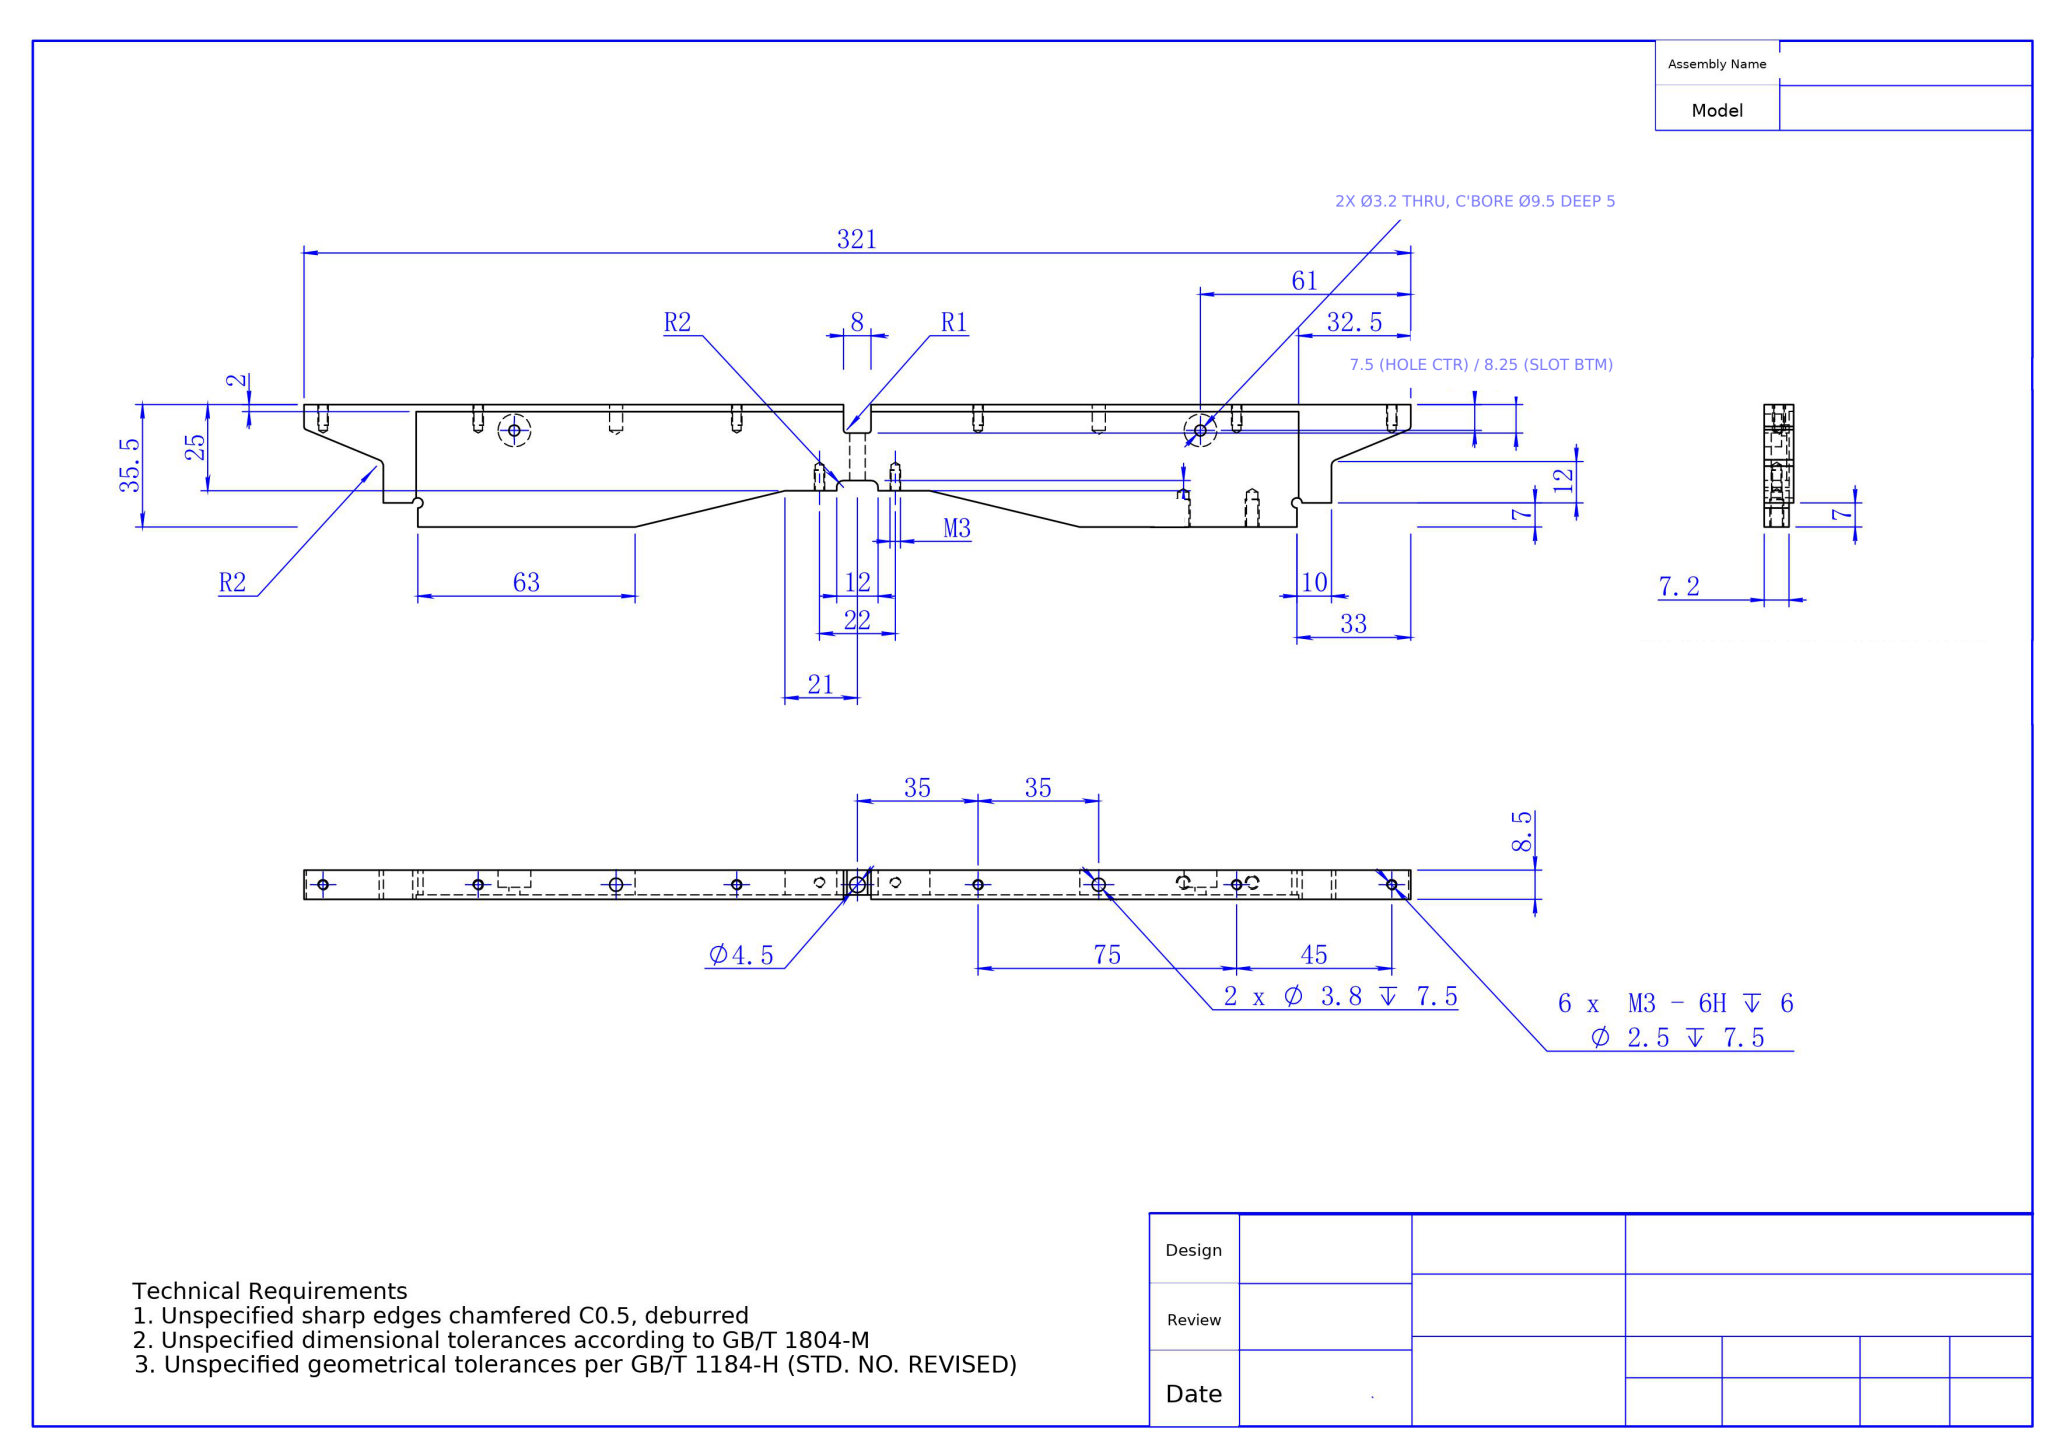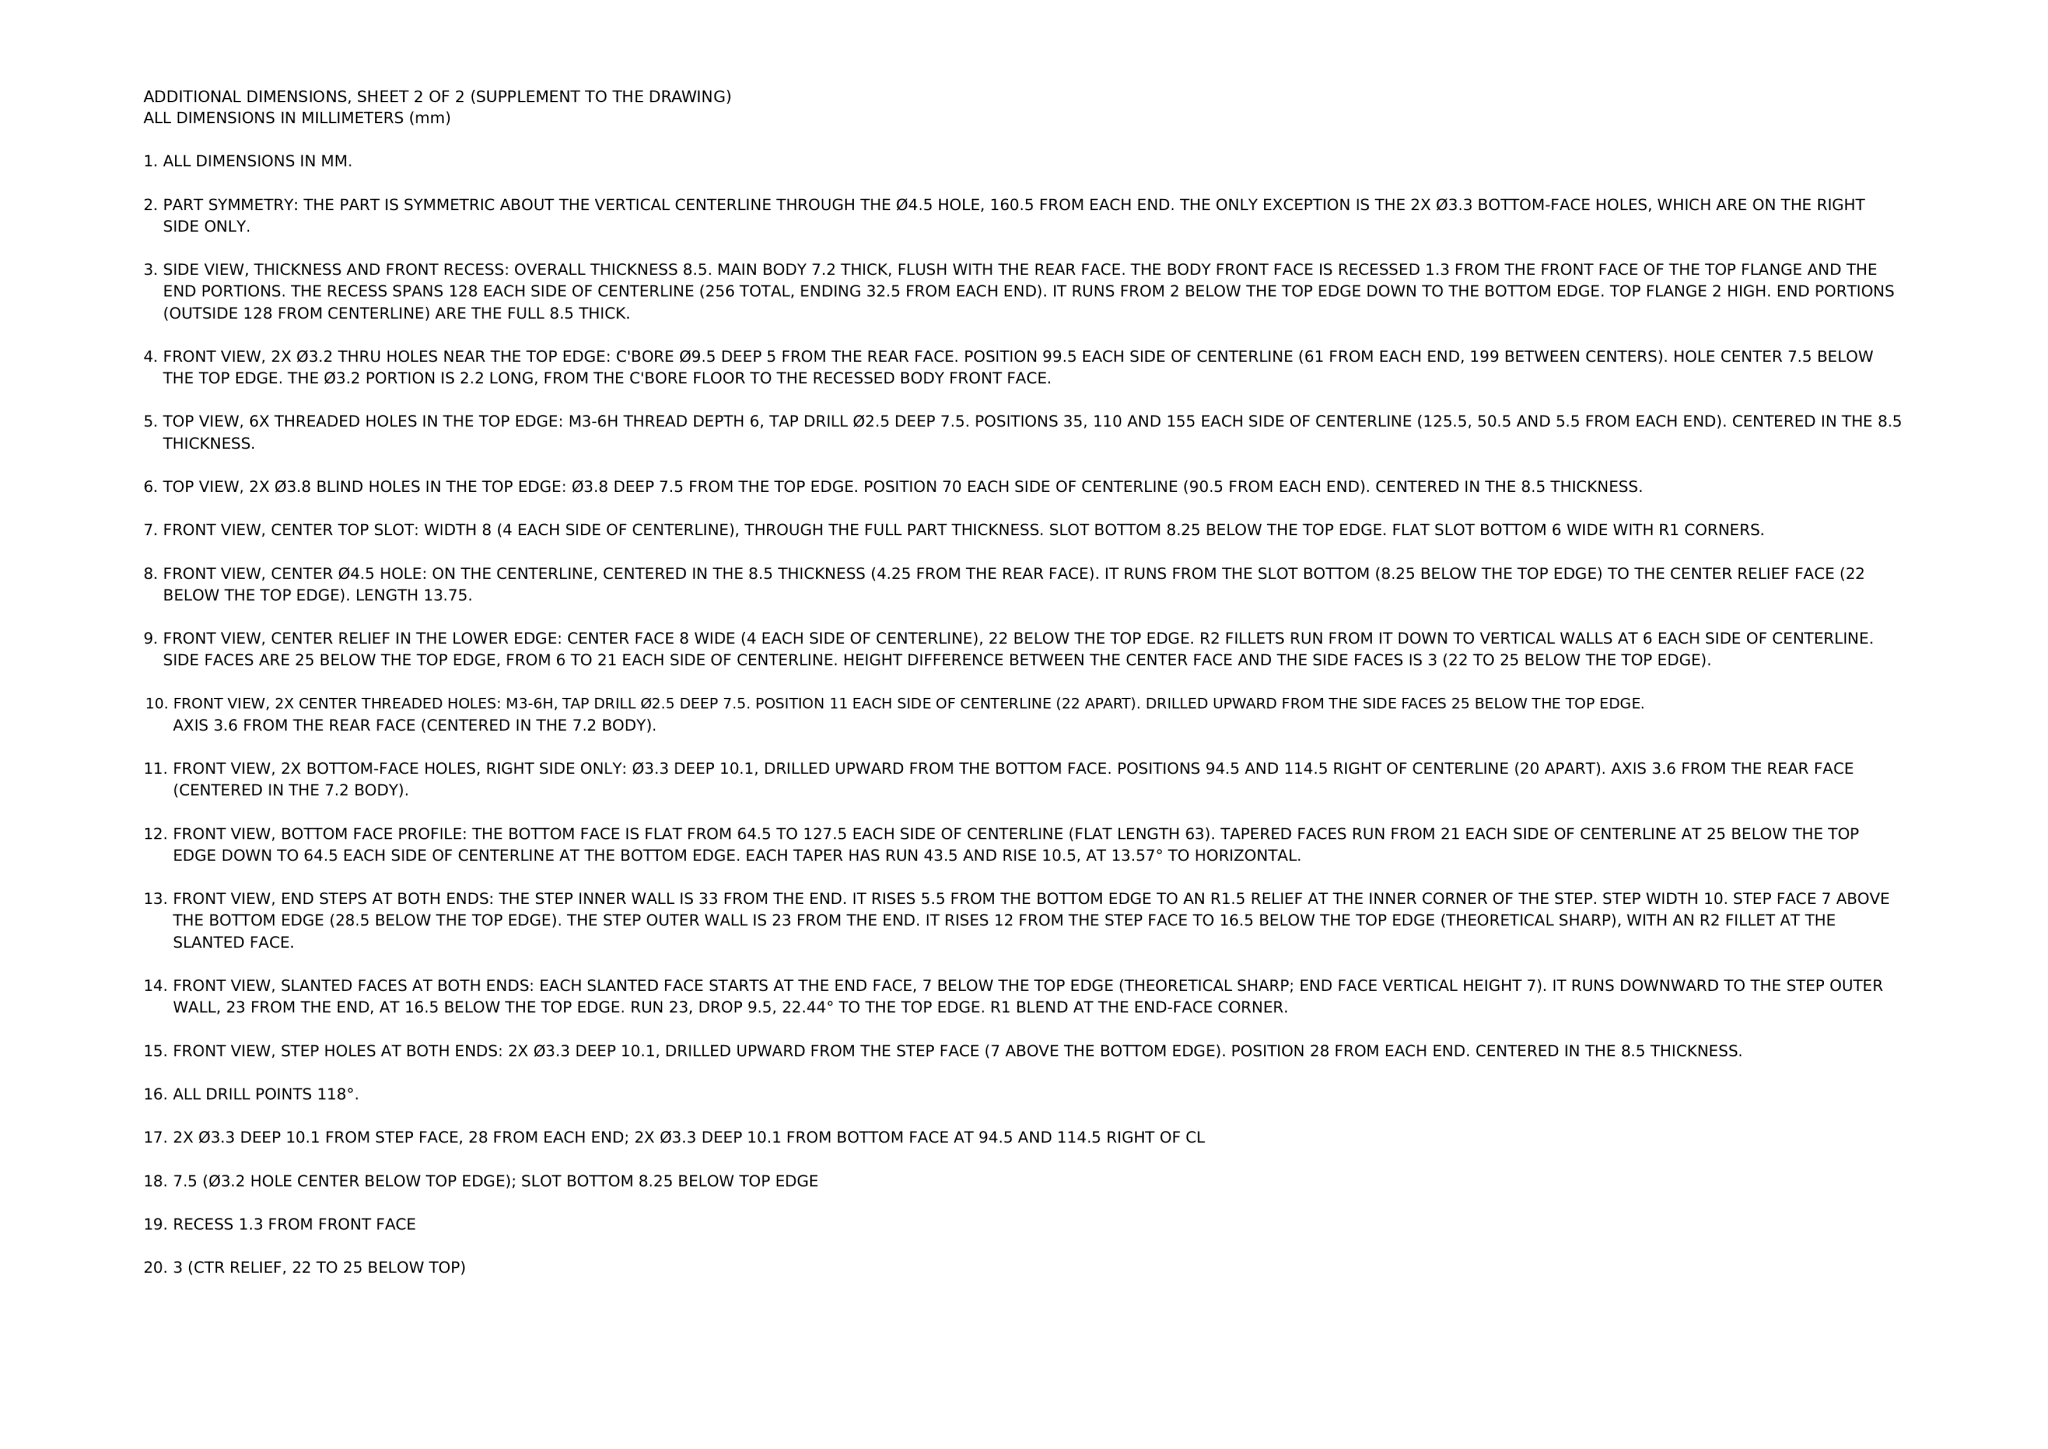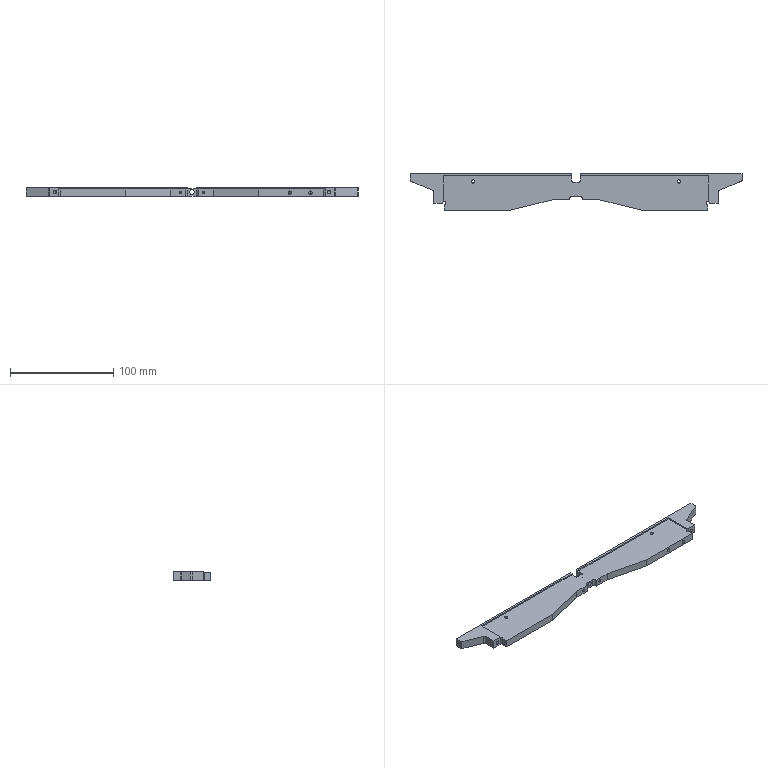Part | NX | mm | 1 solid | 111 faces | box 321 x 35.5 x 8.5 mm | volume 66164 mm3 | cylinder 49 | plane 34 | cone 28 | commonest cylinder face diameters 2.5 x16 3.3 x8 9.5 x4 3.8 x4 3.2 x4 4 x4 2 x4 3 x3